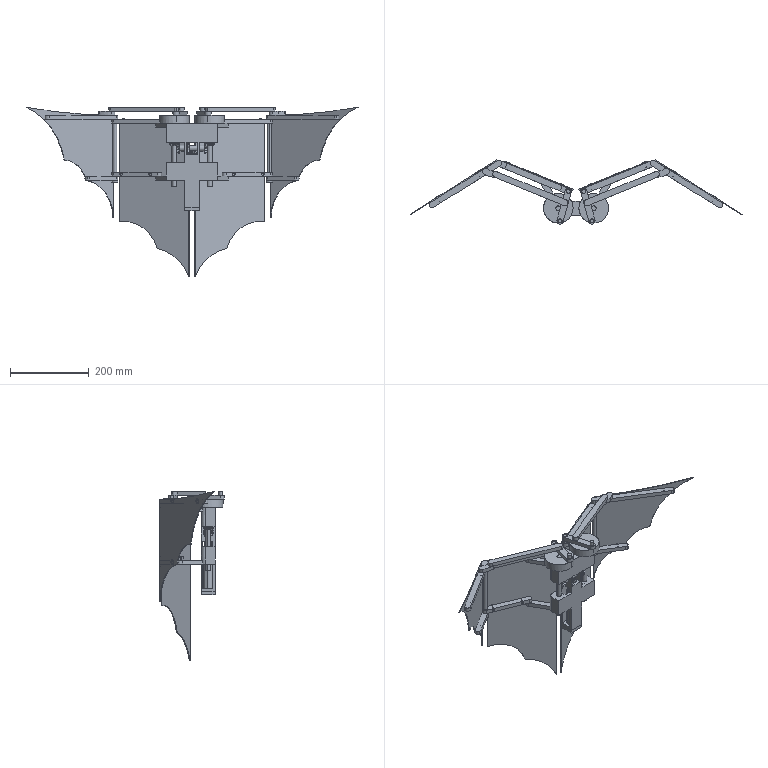Assembly | SolidWorks | mm | 47 component files | 47 solids | 1106 faces | box 842.84 x 162.94 x 430 mm | volume 1387040 mm3 | spline 360 | cylinder 347 | plane 315 | cone 84 | commonest cylinder face diameters 7 x84 12 x82 10 x70 15 x47 20 x20 30 x8 16 x8 25 x6
Bill of materials:
ARocker | 2 |  | Flat bar with a rounded slot shape (straight sides, semicircular ends) and three vertical through-holes: one at each end and one between them.
BevelGearNew | 6 |  | Bevel-type gear: ring of straight teeth on a cone around a large plain central bore.
BRocker(Left) | 1 |  | Flat link bar with rounded ends: a through-hole at one end, a tall cylindrical pin standing up from the other end, and a shorter pin pointing down near the middle.
BRocker(Right) | 1 |  | Flat link bar with rounded ends: a through-hole at one end, an upward cylindrical pin at the other end, and a shorter downward pin part-way along.
CRocker | 2 |  | Flat bar with rounded ends and a short cylindrical pin under each end, both on the same side.
DRocker(Left) | 1 |  | L-shaped part: long flat bar with rounded ends, a long thin rod hanging straight down from one end, and a curved side lug with a through-hole and a short raised boss near that end.
DRocker(Right) | 1 |  | L-shaped part similar to unnamed part, possibly mirrored: flat bar with a downward rod at one end, a curved side lug with a through-hole, a short raised boss, two small cross-holes in the bar, and a notch near the rod tip.
ERocker(Left) | 2 |  | Flat bar with rounded ends: a vertical through-hole at one end, a short cylindrical pin pointing down at the other end, and two cross-holes through the side faces.
FixedWingPin | 14 |  | Headed cylindrical pin: a plain solid cylindrical shank with a thin, flat, larger-diameter disc head at one end.
FRocker | 2 |  | Flat bar with rounded ends, a keyed bore at one end (round hole with a rectangular notch), a plain other end, and one cross-hole in the side face.
GearBushing | 1 |  | Plain cylindrical sleeve or tube with a fairly thick wall; its length is a little less than its outside diameter.
GearShaft | 1 |  | Stepped solid cylindrical pin: a long plain shank with a short wider collar near one end, then a short stub beyond the collar.
InnerWing | 2 |  | Thin flat plate with a rectangular upper portion and a lower edge cut by two adjoining concave arcs, giving a scalloped, tapering lower end; four small through-holes in the upper portion.
MainAxis | 2 |  | Plain, slender solid cylindrical rod with flat ends and constant diameter.
MainBody | 1 |  | Bracket made of two parallel rectangular blocks joined by a central vertical rectangular member with open windows. Each block has two thin flat arms that splay outward in a V shape and end in rounded tips with holes.
Motor | 1 |  | Stepped cylindrical shaft: a large-diameter main body, then a shorter reduced-diameter section with a series of circumferential grooves, ending in a smaller plain cylindrical pin.
MotorCover | 1 |  | Square flat block with a single cylindrical boss on its top face.
OuterWing | 2 |  | Thin flat plate shaped like a curved triangle or wing: a gently curved top edge, one straight side, and a long concave side broken by two scallop arcs. Three small through-holes.
RetainingRing | 2 |  | Plain thick ring (annulus) with a concentric through-bore and flat parallel faces.
Turntable | 2 |  | Circular disk with a central through-hole, a smaller concentric hub on one face, and a single off-centre cylindrical pin standing up from the other face near the rim.
Mates:
1. concentric | MainAxis-1 face at (-69.375, -67.172, -52.818) dir (0, 0, -1) r 6 | Turntable-2 face at (-69.375, -67.172, 107.182) dir (0, 0, 1) r 6
2. coincident | MainAxis-1 face at (-69.375, -67.172, 127.182) dir (0, 0, 1) | Turntable-2 face at (-69.375, -67.172, 127.182) dir (0, 0, 1)
3. concentric | MainAxis-1 face at (-69.375, -67.172, -52.818) dir (0, 0, -1) r 6 | MainBody-2 face at (-69.375, -67.172, 57.182) dir (0, 0, 1) r 6
4. coincident | Turntable-2 face at (-69.375, -67.172, 102.182) dir (0, 0, -1) | MainBody-2 face at (-79.375, -59.672, 102.182) dir (0, 0, 1)
5. concentric | Turntable-2 face at (-64.791, -99.347, 147.182) dir (0, 0, -1) r 5 | ARocker-2 edge at (-64.791, -99.347, 137.182) dir (0, 0, 1) r 5
6. coincident | Turntable-2 face at (-69.375, -67.172, 127.182) dir (0, 0, 1) | ARocker-2 face at (-64.791, -99.347, 127.182) dir (0, 0, -1)
7. concentric | MainBody-2 face at (-109.066, 2.287, 97.182) dir (0, 0, 1) r 5 | BRocker(Left)-2 face at (-109.066, 2.287, 97.182) dir (0, 0, 1) r 5
8. coincident | MainBody-2 face at (-24.375, -67.172, 107.182) dir (0, 0, 1) | BRocker(Left)-2 face at (-56.396, -122.271, 107.182) dir (0, 0, -1)
9. concentric | ARocker-2 face at (-44.233, -24.105, 137.182) dir (0, 0, -1) r 5 | BRocker(Left)-2 face at (-44.233, -24.105, 137.182) dir (0, 0, -1) r 5
10. concentric | ARocker-2 face at (-52.139, -53.045, 137.182) dir (0, 0, -1) r 5 | CRocker-2 face at (-52.139, -53.045, 127.182) dir (0, 0, 1) r 5
11. coincident | ARocker-2 face at (-64.791, -99.347, 137.182) dir (0, 0, 1) | CRocker-2 face at (-51.412, -104.322, 137.182) dir (0, 0, -1)
12. concentric | BRocker(Left)-2 face at (-220.21, 47.531, 107.182) dir (0, 0, 1) r 5 | DRocker(Left)-2 face at (-220.21, 47.531, -42.818) dir (0, 0, 1) r 5
13. coincident | BRocker(Left)-2 face at (-56.396, -122.271, 117.182) dir (0, 0, 1) | DRocker(Left)-2 face at (-25.577, -85.832, 117.182) dir (0, 0, -1)
14. concentric | CRocker-2 face at (-228.043, 18.773, 127.182) dir (0, 0, 1) r 5 | DRocker(Left)-2 face at (-228.043, 18.773, 137.182) dir (0, 0, -1) r 5
15. concentric | ARocker-4 face at (3.389, -53.045, 137.182) dir (0, 0, -1) r 5 | CRocker-4 face at (3.389, -53.045, 127.182) dir (0, 0, 1) r 5
16. coincident | CRocker-2 face at (-51.412, -104.322, 147.182) dir (0, 0, 1) | CRocker-4 face at (215.701, -17.342, 147.182) dir (0, 0, 1)
17. concentric | ARocker-4 face at (-4.518, -24.105, 137.182) dir (0, 0, -1) r 5 | BRocker(Right)-1 face at (-4.518, -24.105, 137.182) dir (0, 0, -1) r 5
18. coincident | ARocker-4 face at (16.04, -99.347, 137.182) dir (0, 0, 1) | BRocker(Right)-1 face at (-4.518, -24.105, 137.182) dir (0, 0, 1)
19. concentric | MainBody-2 face at (60.316, 2.287, 97.182) dir (0, 0, 1) r 5 | BRocker(Right)-1 face at (60.316, 2.287, 97.182) dir (0, 0, 1) r 5
20. concentric | BRocker(Right)-1 face at (171.46, 47.531, 107.182) dir (0, 0, 1) r 5 | DRocker(Right)-1 face at (171.46, 47.531, -42.818) dir (0, 0, 1) r 5
21. concentric | CRocker-4 face at (179.293, 18.773, 127.182) dir (0, 0, 1) r 5 | DRocker(Right)-1 face at (179.293, 18.773, 137.182) dir (0, 0, -1) r 5
22. coincident | CRocker-4 face at (215.701, -17.342, 137.182) dir (0, 0, -1) | DRocker(Right)-1 face at (205.391, 26.35, 137.182) dir (0, 0, 1)
23. concentric | MainBody-2 face at (20.625, -67.172, 57.182) dir (0, 0, 1) r 6 | MainAxis-2 face at (20.625, -67.172, -52.818) dir (0, 0, -1) r 6
24. coincident | MainBody-2 face at (-43.375, -49.672, 22.182) dir (-1, 0, 0) | GearShaft-4 face at (-43.375, -67.172, 42.982) dir (1, 0, 0)
25. concentric | GearShaft-4 face at (12.125, -67.172, 42.982) dir (-1, 0, 0) r 6 | GearBushing-2 face at (6.125, -67.172, 42.982) dir (-1, 0, 0) r 6
26. coincident | MainBody-2 face at (-5.375, -49.672, 22.182) dir (1, 0, 0) | GearBushing-2 face at (-5.375, -67.172, 42.982) dir (-1, 0, 0)
27. concentric | MainAxis-2 face at (20.625, -67.172, -52.818) dir (0, 0, -1) r 6 | Turntable-9 face at (20.625, -67.172, 107.182) dir (0, 0, 1) r 6
28. coincident | MainBody-2 face at (-24.375, -67.172, 107.182) dir (0, 0, 1) | Turntable-9 face at (20.625, -67.172, 107.182) dir (0, 0, -1)
29. concentric | ARocker-4 face at (16.04, -99.347, 137.182) dir (0, 0, -1) r 5 | Turntable-9 face at (16.04, -99.347, 147.182) dir (0, 0, -1) r 5
30. coincident | MainBody-2 face at (-24.375, -67.172, 22.182) dir (0, 0, -1) | Motor-2 face at (-24.375, -67.172, 22.182) dir (0, 0, 1)
31. concentric | MainBody-2 face at (60.316, 2.287, -37.818) dir (0, 0, 1) r 5 | ERocker(Left)-3 face at (60.316, 2.287, -37.818) dir (0, 0, 1) r 5
32. coincident | MainBody-2 face at (60.316, 2.287, -27.818) dir (0, 0, 1) | ERocker(Left)-3 face at (-64.373, 54.646, -27.818) dir (0, 0, -1)
33. concentric | DRocker(Right)-1 face at (171.46, 47.531, -42.818) dir (0, 0, 1) r 5 | ERocker(Left)-3 face at (171.46, 47.531, -27.818) dir (0, 0, 1) r 5
34. concentric | MainBody-2 face at (-109.066, 2.287, -37.818) dir (0, 0, 1) r 5 | ERocker(Left)-4 face at (-109.066, 2.287, -37.818) dir (0, 0, 1) r 5
35. coincident | MainBody-2 face at (-24.375, -67.172, -37.818) dir (0, 0, -1) | ERocker(Left)-4 face at (-56.396, -122.271, -37.818) dir (0, 0, -1)
36. concentric | DRocker(Left)-2 face at (-220.21, 47.531, -42.818) dir (0, 0, 1) r 5 | ERocker(Left)-4 face at (-220.21, 47.531, -27.818) dir (0, 0, 1) r 5
37. concentric | DRocker(Right)-1 face at (171.46, 47.531, -42.818) dir (0, 0, 1) r 5 | FRocker-1 face at (171.46, 47.531, -27.818) dir (0, 0, -1) r 5
38. coincident | ERocker(Left)-3 face at (-64.373, 54.646, -27.818) dir (0, 0, -1) | FRocker-1 face at (205.792, 280.96, -27.818) dir (0, 0, 1)
39. coincident | DRocker(Right)-1 face at (170.401, 45.835, -27.818) dir (0.5295, 0.8483, 0) | FRocker-1 face at (90.25, 95.868, -27.818) dir (-0.5295, -0.8483, 0)
40. concentric | DRocker(Right)-1 face at (221.033, 13.638, 122.182) dir (0.5295, 0.8483, 0) r 3.5 | OuterWing-2 face at (226.328, 22.121, 122.182) dir (0.5295, 0.8483, 0) r 3.5
41. coincident | DRocker(Right)-1 face at (95.28, 103.927, 127.182) dir (0.5295, 0.8483, 0) | OuterWing-2 face at (95.28, 103.927, -37.818) dir (-0.5295, -0.8483, 0)
42. concentric | DRocker(Left)-2 face at (-220.21, 47.531, -42.818) dir (0, 0, 1) r 5 | FRocker-3 face at (-220.21, 47.531, -37.818) dir (0, 0, 1) r 5
43. coincident | ERocker(Left)-4 face at (-56.396, -122.271, -27.818) dir (0, 0, -1) | FRocker-3 face at (-254.541, 280.96, -27.818) dir (0, 0, 1)
44. coincident | DRocker(Left)-2 face at (-229.752, 43.932, -27.818) dir (0.5295, -0.8483, 0) | FRocker-3 face at (-141.118, 99.261, -37.818) dir (-0.5295, 0.8483, 0)
45. concentric | DRocker(Left)-2 edge at (-275.079, 22.121, 122.182) dir (-0.5295, 0.8483, 0) r 3.5 | OuterWing-3 face at (-276.138, 23.818, 122.182) dir (0.5295, -0.8483, 0) r 3.5
46. concentric | OuterWing-3 face at (-276.138, 23.818, -32.818) dir (0.5295, -0.8483, 0) r 3.5 | FRocker-3 face at (-269.784, 13.639, -32.818) dir (-0.5295, 0.8483, 0) r 3.5
47. coincident | OuterWing-3 face at (-144.031, 103.926, -37.818) dir (0.5295, -0.8483, 0) | FRocker-3 face at (-144.031, 103.926, -37.818) dir (-0.5295, 0.8483, 0)
48. concentric | MainBody-2 face at (-24.375, -67.172, 2.182) dir (0, 0, -1) r 12.5 | MotorCover-1 face at (-24.375, -67.172, -99.818) dir (0, 0, -1) r 12.5
49. coincident | MainBody-2 face at (-24.375, -67.172, -107.818) dir (0, 0, -1) | MotorCover-1 face at (-24.375, -67.172, -107.818) dir (0, 0, 1)
50. coincident | MainAxis-2 face at (20.625, -67.172, 127.182) dir (0, 0, 1) | Turntable-9 face at (20.625, -67.172, 127.182) dir (0, 0, 1)
51. concentric | ARocker-4 face at (16.04, -99.347, 137.182) dir (0, 0, -1) r 5 | Turntable-9 face at (16.04, -99.347, 147.182) dir (0, 0, -1) r 5
52. concentric | MainBody-2 face at (-24.375, -67.172, 2.182) dir (0, 0, -1) r 12.5 | Motor-2 face at (-24.375, -67.172, -99.818) dir (0, 0, 1) r 12.5
53. concentric | MainBody-2 face at (67.816, -67.172, 42.982) dir (-1, 0, 0) r 6 | GearShaft-4 face at (12.125, -67.172, 42.982) dir (-1, 0, 0) r 6
54. coincident | ARocker-4 face at (16.04, -99.347, 137.182) dir (0, 0, 1) | CRocker-4 face at (215.701, -17.342, 137.182) dir (0, 0, -1)
55. concentric | Motor-2 face at (-24.375, -67.172, 35.682) dir (0, 0, -1) r 6 | BevelGearNew-1 face at (-24.375, -67.172, 41.783) dir (0, 0, -1) r 6
56. coincident | MainBody-2 face at (67.818, -49.672, 27.682) dir (0, 0, 1) | BevelGearNew-1 face at (-24.375, -67.172, 27.682) dir (0, 0, -1)
57. concentric | GearShaft-4 face at (12.125, -67.172, 42.982) dir (-1, 0, 0) r 6 | BevelGearNew-12 face at (-24.274, -67.172, 42.982) dir (-1, 0, 0) r 6
58. coincident | MainBody-2 face at (-38.375, -49.672, 22.182) dir (1, 0, 0) | BevelGearNew-12 face at (-38.375, -67.172, 42.982) dir (-1, 0, 0)
59. concentric | GearShaft-4 face at (12.125, -67.172, 42.982) dir (-1, 0, 0) r 6 | BevelGearNew-14 face at (20.226, -67.172, 42.982) dir (-1, 0, 0) r 6
60. coincident | GearBushing-2 face at (6.125, -67.172, 42.982) dir (1, 0, 0) | BevelGearNew-14 face at (6.125, -67.172, 42.982) dir (-1, 0, 0)
61. concentric | MainAxis-2 face at (20.625, -67.172, -52.818) dir (0, 0, 1) r 6 | BevelGearNew-16 face at (20.625, -67.172, 43.081) dir (0, 0, 1) r 6
62. coincident | MainBody-2 face at (-79.375, -59.672, 57.182) dir (0, 0, -1) | BevelGearNew-16 face at (20.625, -67.172, 57.182) dir (0, 0, 1)
63. concentric | MainAxis-1 face at (-69.375, -67.172, -52.818) dir (0, 0, 1) r 6 | BevelGearNew-18 face at (-69.375, -67.172, 43.081) dir (0, 0, 1) r 6
64. coincident | MainBody-2 face at (-79.375, -59.672, 57.182) dir (0, 0, -1) | BevelGearNew-18 face at (-69.375, -67.172, 57.182) dir (0, 0, 1)
65. concentric | GearShaft-4 face at (12.125, -67.172, 42.982) dir (-1, 0, 0) r 6 | BevelGearNew-20 face at (-68.976, -67.172, 42.982) dir (1, 0, 0) r 6
66. coincident | GearShaft-4 face at (-54.875, -67.172, 42.982) dir (-1, 0, 0) | BevelGearNew-20 face at (-54.875, -67.172, 42.982) dir (1, 0, 0)
67. gear | BevelGearNew-14 face at (15.878, -67.172, 42.982) dir (1, 0, 0) r 902.708 | BevelGearNew-16 face at (20.625, -67.172, 47.43) dir (0, 0, -1) r 902.708
68. gear | BevelGearNew-1 face at (-24.375, -67.172, 37.435) dir (0, 0, 1) r 902.708 | BevelGearNew-12 face at (-28.622, -67.172, 42.982) dir (1, 0, 0) r 902.708
69. gear | BevelGearNew-20 face at (-64.628, -67.172, 42.982) dir (-1, 0, 0) r 902.708 | BevelGearNew-18 face at (-69.375, -67.172, 47.43) dir (0, 0, -1) r 902.708
70. concentric | ERocker(Left)-4 face at (-130.795, 1.955, -22.818) dir (0.377, 0.9262, 0) r 3.5 | InnerWing-1 face at (-124.763, 16.774, -22.818) dir (0.377, 0.9262, 0) r 3.5
71. concentric | ERocker(Left)-4 face at (-204.891, 32.118, -22.818) dir (0.377, 0.9262, 0) r 3.5 | InnerWing-1 face at (-198.859, 46.937, -22.818) dir (0.377, 0.9262, 0) r 3.5
72. coincident | ERocker(Left)-4 face at (-17.559, -26.866, -17.818) dir (0.377, 0.9262, 0) | InnerWing-1 face at (-18.038, -26.671, 107.182) dir (-0.377, -0.9262, 0)
73. concentric | BRocker(Left)-2 face at (-63.699, -18.88, 112.182) dir (0.377, 0.9262, 0) r 3.5 | InnerWing-1 face at (-59.929, -9.618, 112.182) dir (0.377, 0.9262, 0) r 3.5
74. concentric | BRocker(Right)-1 face at (14.948, -18.88, 112.182) dir (-0.377, 0.9262, 0) r 3.5 | InnerWing-3 face at (10.424, -7.766, 112.182) dir (0.377, -0.9262, 0) r 3.5
75. coincident | BRocker(Right)-1 face at (-31.192, -26.866, 117.182) dir (-0.377, 0.9262, 0) | InnerWing-3 face at (-30.713, -26.671, 107.182) dir (0.377, -0.9262, 0)
76. concentric | ERocker(Left)-3 face at (149.731, 47.863, -22.818) dir (-0.377, 0.9262, 0) r 3.5 | InnerWing-3 face at (149.354, 48.789, -22.818) dir (0.377, -0.9262, 0) r 3.5
77. concentric | OuterWing-3 face at (-377.933, -39.726, 122.182) dir (0.5295, -0.8483, 0) r 3.5 | FixedWingPin-2 face at (-371.579, -49.905, 122.182) dir (-0.5295, 0.8483, 0) r 3.5
78. coincident | OuterWing-3 face at (-145.09, 105.623, -37.818) dir (-0.5295, 0.8483, 0) | FixedWingPin-2 face at (-377.933, -39.726, 122.182) dir (0.5295, -0.8483, 0)
79. concentric | DRocker(Left)-2 face at (-269.784, 13.639, 122.182) dir (-0.5295, 0.8483, 0) r 3.5 | FixedWingPin-3 face at (-269.784, 13.639, 122.182) dir (-0.5295, 0.8483, 0) r 3.5
80. coincident | OuterWing-3 face at (-145.09, 105.623, -37.818) dir (-0.5295, 0.8483, 0) | FixedWingPin-3 face at (-276.138, 23.818, 122.182) dir (0.5295, -0.8483, 0)
81. concentric | FRocker-3 face at (-269.784, 13.639, -32.818) dir (-0.5295, 0.8483, 0) r 3.5 | FixedWingPin-5 face at (-269.784, 13.639, -32.818) dir (-0.5295, 0.8483, 0) r 3.5
82. coincident | OuterWing-3 face at (-145.09, 105.623, -37.818) dir (-0.5295, 0.8483, 0) | FixedWingPin-5 face at (-276.138, 23.818, -32.818) dir (0.5295, -0.8483, 0)
83. concentric | ERocker(Left)-4 face at (-204.891, 32.118, -22.818) dir (0.377, 0.9262, 0) r 3.5 | FixedWingPin-7 face at (-202.629, 37.675, -22.818) dir (0.377, 0.9262, 0) r 3.5
84. coincident | InnerWing-1 face at (-17.284, -24.819, 107.182) dir (0.377, 0.9262, 0) | FixedWingPin-7 face at (-198.105, 48.789, -22.818) dir (-0.377, -0.9262, 0)
85. concentric | InnerWing-1 face at (-198.859, 46.937, 112.182) dir (0.377, 0.9262, 0) r 3.5 | FixedWingPin-9 face at (-202.629, 37.675, 112.182) dir (0.377, 0.9262, 0) r 3.5
86. coincident | InnerWing-1 face at (-17.284, -24.819, 107.182) dir (0.377, 0.9262, 0) | FixedWingPin-9 face at (-198.105, 48.789, 112.182) dir (-0.377, -0.9262, 0)
87. concentric | InnerWing-1 face at (-59.929, -9.618, 112.182) dir (0.377, 0.9262, 0) r 3.5 | FixedWingPin-11 face at (-63.699, -18.88, 112.182) dir (0.377, 0.9262, 0) r 3.5
88. coincident | InnerWing-1 face at (-17.284, -24.819, 107.182) dir (0.377, 0.9262, 0) | FixedWingPin-11 face at (-59.175, -7.766, 112.182) dir (-0.377, -0.9262, 0)
89. concentric | InnerWing-1 face at (-124.763, 16.774, -22.818) dir (0.377, 0.9262, 0) r 3.5 | FixedWingPin-13 face at (-128.533, 7.512, -22.818) dir (0.377, 0.9262, 0) r 3.5
90. coincident | InnerWing-1 face at (-17.284, -24.819, 107.182) dir (0.377, 0.9262, 0) | FixedWingPin-13 face at (-124.009, 18.627, -22.818) dir (-0.377, -0.9262, 0)
91. concentric | BRocker(Right)-1 face at (14.948, -18.88, 112.182) dir (-0.377, 0.9262, 0) r 3.5 | FixedWingPin-15 face at (14.948, -18.88, 112.182) dir (-0.377, 0.9262, 0) r 3.5
92. coincident | InnerWing-3 face at (-31.467, -24.819, 107.182) dir (-0.377, 0.9262, 0) | FixedWingPin-15 face at (10.424, -7.766, 112.182) dir (0.377, -0.9262, 0)
93. concentric | ERocker(Left)-3 face at (75.635, 17.7, -22.818) dir (-0.377, 0.9262, 0) r 3.5 | FixedWingPin-17 face at (79.782, 7.512, -22.818) dir (-0.377, 0.9262, 0) r 3.5
94. coincident | InnerWing-3 face at (-31.467, -24.819, 107.182) dir (-0.377, 0.9262, 0) | FixedWingPin-17 face at (75.258, 18.627, -22.818) dir (0.377, -0.9262, 0)
95. concentric | ERocker(Left)-3 face at (149.731, 47.863, -22.818) dir (-0.377, 0.9262, 0) r 3.5 | FixedWingPin-19 face at (153.878, 37.675, -22.818) dir (-0.377, 0.9262, 0) r 3.5
96. coincident | InnerWing-3 face at (-31.467, -24.819, 107.182) dir (-0.377, 0.9262, 0) | FixedWingPin-19 face at (149.354, 48.789, -22.818) dir (0.377, -0.9262, 0)
97. concentric | BRocker(Right)-1 face at (153.878, 37.675, 112.182) dir (-0.377, 0.9262, 0) r 3.5 | FixedWingPin-22 face at (153.878, 37.675, 112.182) dir (-0.377, 0.9262, 0) r 3.5
98. coincident | InnerWing-3 face at (-31.467, -24.819, 107.182) dir (-0.377, 0.9262, 0) | FixedWingPin-22 face at (149.354, 48.789, 112.182) dir (0.377, -0.9262, 0)
99. concentric | DRocker(Right)-1 face at (221.033, 13.638, 122.182) dir (0.5295, 0.8483, 0) r 3.5 | FixedWingPin-24 face at (221.033, 13.638, 122.182) dir (0.5295, 0.8483, 0) r 3.5
100. coincident | OuterWing-2 face at (96.339, 105.623, -37.818) dir (0.5295, 0.8483, 0) | FixedWingPin-24 face at (227.388, 23.818, 122.182) dir (-0.5295, -0.8483, 0)
101. concentric | DRocker(Right)-1 face at (322.828, -49.906, 122.182) dir (0.5295, 0.8483, 0) r 3.5 | FixedWingPin-26 face at (322.828, -49.906, 122.182) dir (0.5295, 0.8483, 0) r 3.5
102. coincident | OuterWing-2 face at (96.339, 105.623, -37.818) dir (0.5295, 0.8483, 0) | FixedWingPin-26 face at (329.182, -39.727, 122.182) dir (-0.5295, -0.8483, 0)
103. concentric | FRocker-1 face at (221.033, 13.638, -32.818) dir (0.5295, 0.8483, 0) r 3.5 | FixedWingPin-28 face at (221.033, 13.638, -32.818) dir (0.5295, 0.8483, 0) r 3.5
104. coincident | OuterWing-2 face at (96.339, 105.623, -37.818) dir (0.5295, 0.8483, 0) | FixedWingPin-28 face at (227.388, 23.818, -32.818) dir (-0.5295, -0.8483, 0)
105. concentric | DRocker(Right)-1 face at (171.46, 47.531, -42.818) dir (0, 0, 1) r 5 | RetainingRing-2 face at (171.46, 47.531, -42.818) dir (0, 0, 1) r 5
106. coincident | FRocker-1 face at (205.792, 280.96, -37.818) dir (0, 0, -1) | RetainingRing-2 face at (171.46, 47.531, -37.818) dir (0, 0, 1)
107. concentric | DRocker(Left)-2 face at (-220.21, 47.531, -42.818) dir (0, 0, 1) r 5 | RetainingRing-3 face at (-220.21, 47.531, -42.818) dir (0, 0, 1) r 5
108. coincident | FRocker-3 face at (-254.541, 280.96, -37.818) dir (0, 0, -1) | RetainingRing-3 face at (-220.21, 47.531, -37.818) dir (0, 0, 1)